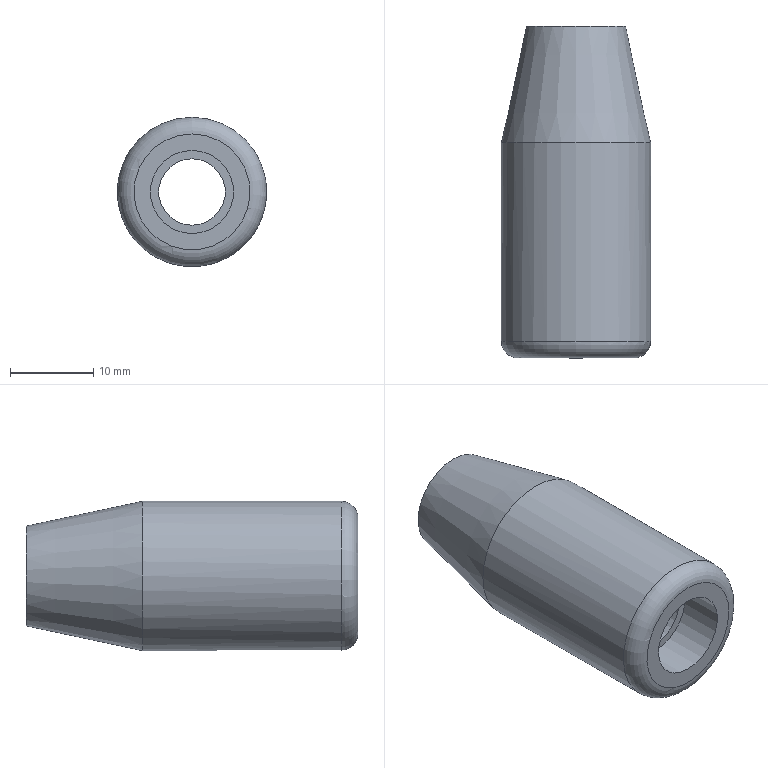Component | NX | HANDLE | 1 solid | 8 faces | box 17.95 x 39.9 x 17.95 mm | volume 6847 mm3 | plane 3 | cylinder 3 | cone 1 | torus 1 | commonest cylinder face diameters 17.952 x1 8 x1 10 x1
STEP:
#1=CARTESIAN_POINT('',(0.,0.,0.));
#2=DIRECTION('',(0.,0.,1.));
#3=DIRECTION('',(1.,0.,0.));
#4=AXIS2_PLACEMENT_3D('',#1,#2,#3);
#5=CARTESIAN_POINT('',(-0.,-194.8,71.));
#6=VERTEX_POINT('',#5);
#7=CARTESIAN_POINT('',(-0.,-194.8,67.));
#8=DIRECTION('',(0.,1.,0.));
#9=DIRECTION('',(0.,0.,1.));
#10=AXIS2_PLACEMENT_3D('',#7,#8,#9);
#11=CIRCLE('',#10,4.);
#12=CARTESIAN_POINT('',(-0.,-194.8,67.));
#13=DIRECTION('',(0.,1.,0.));
#14=DIRECTION('',(0.,0.,1.));
#15=AXIS2_PLACEMENT_3D('',#12,#13,#14);
#16=PLANE('',#15);
#17=CARTESIAN_POINT('',(0.,0.));
#18=DIRECTION('',(1.,0.));
#19=AXIS2_PLACEMENT_2D('',#17,#18);
#20=CIRCLE('',#19,4.);
#21=(GEOMETRIC_REPRESENTATION_CONTEXT(2)PARAMETRIC_REPRESENTATION_CONTEXT()REPRESENTATION_CONTEXT('',''));
#22=DEFINITIONAL_REPRESENTATION('',(#20),#21);
#23=PCURVE('',#16,#22);
#24=CARTESIAN_POINT('',(-0.,-188.739,67.));
#25=DIRECTION('',(0.,1.,0.));
#26=DIRECTION('',(0.,0.,1.));
#27=AXIS2_PLACEMENT_3D('',#24,#25,#26);
#28=CYLINDRICAL_SURFACE('',#27,4.);
#29=CARTESIAN_POINT('',(0.,-6.061));
#30=DIRECTION('',(1.,0.));
#31=VECTOR('',#30,1.);
#32=LINE('',#29,#31);
#33=(GEOMETRIC_REPRESENTATION_CONTEXT(2)PARAMETRIC_REPRESENTATION_CONTEXT()REPRESENTATION_CONTEXT('',''));
#34=DEFINITIONAL_REPRESENTATION('',(#32),#33);
#35=PCURVE('',#28,#34);
#36=SURFACE_CURVE('',#11,(#23,#35),.PCURVE_S1.);
#37=EDGE_CURVE('',#6,#6,#36,.T.);
#38=ORIENTED_EDGE('',*,*,#37,.F.);
#39=EDGE_LOOP('',(#38));
#40=FACE_BOUND('',#39,.T.);
#41=CARTESIAN_POINT('',(-0.,-194.8,61.));
#42=VERTEX_POINT('',#41);
#43=CARTESIAN_POINT('',(-0.,-194.8,67.));
#44=DIRECTION('',(0.,-1.,0.));
#45=DIRECTION('',(0.,0.,-1.));
#46=AXIS2_PLACEMENT_3D('',#43,#44,#45);
#47=CIRCLE('',#46,6.);
#48=CARTESIAN_POINT('',(-6.,0.));
#49=CARTESIAN_POINT('',(-6.,10.392));
#50=CARTESIAN_POINT('',(3.,5.196));
#51=CARTESIAN_POINT('',(12.,0.));
#52=CARTESIAN_POINT('',(3.,-5.196));
#53=CARTESIAN_POINT('',(-6.,-10.392));
#54=CARTESIAN_POINT('',(-6.,0.));
#55=(BOUNDED_CURVE()B_SPLINE_CURVE(2,(#48,#49,#50,#51,#52,#53,#54),.UNSPECIFIED.,.T.,.F.)B_SPLINE_CURVE_WITH_KNOTS((1,2,2,2,2,1),(-2.094,0.,2.094,4.189,6.283,8.378),.UNSPECIFIED.)CURVE()GEOMETRIC_REPRESENTATION_ITEM()RATIONAL_B_SPLINE_CURVE((1.,0.5,1.,0.5,1.,0.5,1.))REPRESENTATION_ITEM(''));
#56=(GEOMETRIC_REPRESENTATION_CONTEXT(2)PARAMETRIC_REPRESENTATION_CONTEXT()REPRESENTATION_CONTEXT('',''));
#57=DEFINITIONAL_REPRESENTATION('',(#55),#56);
#58=PCURVE('',#16,#57);
#59=CARTESIAN_POINT('',(-0.,-194.8,67.));
#60=DIRECTION('',(0.,-1.,0.));
#61=DIRECTION('',(0.,0.,-1.));
#62=AXIS2_PLACEMENT_3D('',#59,#60,#61);
#63=CONICAL_SURFACE('',#62,6.,0.2094);
#64=CARTESIAN_POINT('',(0.,0.));
#65=DIRECTION('',(1.,0.));
#66=VECTOR('',#65,1.);
#67=LINE('',#64,#66);
#68=(GEOMETRIC_REPRESENTATION_CONTEXT(2)PARAMETRIC_REPRESENTATION_CONTEXT()REPRESENTATION_CONTEXT('',''));
#69=DEFINITIONAL_REPRESENTATION('',(#67),#68);
#70=PCURVE('',#63,#69);
#71=SURFACE_CURVE('',#47,(#58,#70),.PCURVE_S1.);
#72=EDGE_CURVE('',#42,#42,#71,.T.);
#73=ORIENTED_EDGE('',*,*,#72,.F.);
#74=EDGE_LOOP('',(#73));
#75=FACE_BOUND('',#74,.T.);
#76=ADVANCED_FACE('',(#40,#75),#16,.T.);
#77=ORIENTED_EDGE('',*,*,#72,.T.);
#78=CARTESIAN_POINT('',(-0.,-208.8,58.024));
#79=VERTEX_POINT('',#78);
#80=CARTESIAN_POINT('',(-0.,-194.8,61.));
#81=CARTESIAN_POINT('',(-0.,-208.8,58.024));
#82=B_SPLINE_CURVE_WITH_KNOTS('',1,(#80,#81),.UNSPECIFIED.,.F.,.F.,(2,2),(0.,14.313),.PIECEWISE_BEZIER_KNOTS.);
#83=CARTESIAN_POINT('',(6.283,0.));
#84=DIRECTION('',(0.,1.));
#85=VECTOR('',#84,1.);
#86=LINE('',#83,#85);
#87=(GEOMETRIC_REPRESENTATION_CONTEXT(2)PARAMETRIC_REPRESENTATION_CONTEXT()REPRESENTATION_CONTEXT('',''));
#88=DEFINITIONAL_REPRESENTATION('',(#86),#87);
#89=PCURVE('',#63,#88);
#90=CARTESIAN_POINT('',(0.,0.));
#91=DIRECTION('',(0.,1.));
#92=VECTOR('',#91,1.);
#93=LINE('',#90,#92);
#94=(GEOMETRIC_REPRESENTATION_CONTEXT(2)PARAMETRIC_REPRESENTATION_CONTEXT()REPRESENTATION_CONTEXT('',''));
#95=DEFINITIONAL_REPRESENTATION('',(#93),#94);
#96=PCURVE('',#63,#95);
#97=SEAM_CURVE('',#82,(#89,#96),.PCURVE_S1.);
#98=EDGE_CURVE('',#42,#79,#97,.T.);
#99=ORIENTED_EDGE('',*,*,#98,.T.);
#100=CARTESIAN_POINT('',(-0.,-208.8,75.976));
#101=VERTEX_POINT('',#100);
#102=CARTESIAN_POINT('',(-0.,-208.8,67.));
#103=DIRECTION('',(0.,1.,0.));
#104=DIRECTION('',(0.,0.,-1.));
#105=AXIS2_PLACEMENT_3D('',#102,#103,#104);
#106=CIRCLE('',#105,8.976);
#107=CARTESIAN_POINT('',(6.283,14.));
#108=DIRECTION('',(-1.,0.));
#109=VECTOR('',#108,1.);
#110=LINE('',#107,#109);
#111=(GEOMETRIC_REPRESENTATION_CONTEXT(2)PARAMETRIC_REPRESENTATION_CONTEXT()REPRESENTATION_CONTEXT('',''));
#112=DEFINITIONAL_REPRESENTATION('',(#110),#111);
#113=PCURVE('',#63,#112);
#114=CARTESIAN_POINT('',(-0.,-234.7,67.));
#115=DIRECTION('',(0.,1.,0.));
#116=DIRECTION('',(0.,0.,1.));
#117=AXIS2_PLACEMENT_3D('',#114,#115,#116);
#118=CYLINDRICAL_SURFACE('',#117,8.976);
#119=CARTESIAN_POINT('',(3.142,25.9));
#120=DIRECTION('',(1.,0.));
#121=VECTOR('',#120,1.);
#122=LINE('',#119,#121);
#123=(GEOMETRIC_REPRESENTATION_CONTEXT(2)PARAMETRIC_REPRESENTATION_CONTEXT()REPRESENTATION_CONTEXT('',''));
#124=DEFINITIONAL_REPRESENTATION('',(#122),#123);
#125=PCURVE('',#118,#124);
#126=SURFACE_CURVE('',#106,(#113,#125),.PCURVE_S1.);
#127=EDGE_CURVE('',#79,#101,#126,.T.);
#128=ORIENTED_EDGE('',*,*,#127,.T.);
#129=CARTESIAN_POINT('',(-0.,-208.8,67.));
#130=DIRECTION('',(0.,1.,0.));
#131=DIRECTION('',(0.,0.,-1.));
#132=AXIS2_PLACEMENT_3D('',#129,#130,#131);
#133=CIRCLE('',#132,8.976);
#134=CARTESIAN_POINT('',(6.283,14.));
#135=DIRECTION('',(-1.,0.));
#136=VECTOR('',#135,1.);
#137=LINE('',#134,#136);
#138=(GEOMETRIC_REPRESENTATION_CONTEXT(2)PARAMETRIC_REPRESENTATION_CONTEXT()REPRESENTATION_CONTEXT('',''));
#139=DEFINITIONAL_REPRESENTATION('',(#137),#138);
#140=PCURVE('',#63,#139);
#141=CARTESIAN_POINT('',(-3.142,25.9));
#142=DIRECTION('',(1.,0.));
#143=VECTOR('',#142,1.);
#144=LINE('',#141,#143);
#145=(GEOMETRIC_REPRESENTATION_CONTEXT(2)PARAMETRIC_REPRESENTATION_CONTEXT()REPRESENTATION_CONTEXT('',''));
#146=DEFINITIONAL_REPRESENTATION('',(#144),#145);
#147=PCURVE('',#118,#146);
#148=SURFACE_CURVE('',#133,(#140,#147),.PCURVE_S1.);
#149=EDGE_CURVE('',#101,#79,#148,.T.);
#150=ORIENTED_EDGE('',*,*,#149,.T.);
#151=ORIENTED_EDGE('',*,*,#98,.F.);
#152=EDGE_LOOP('',(#77,#99,#128,#150,#151));
#153=FACE_BOUND('',#152,.T.);
#154=ADVANCED_FACE('',(#153),#63,.T.);
#155=CARTESIAN_POINT('',(-0.,-232.7,75.976));
#156=VERTEX_POINT('',#155);
#157=CARTESIAN_POINT('',(-0.,-232.7,67.));
#158=DIRECTION('',(0.,1.,0.));
#159=DIRECTION('',(0.,0.,1.));
#160=AXIS2_PLACEMENT_3D('',#157,#158,#159);
#161=CIRCLE('',#160,8.976);
#162=CARTESIAN_POINT('',(0.,2.));
#163=DIRECTION('',(1.,0.));
#164=VECTOR('',#163,1.);
#165=LINE('',#162,#164);
#166=(GEOMETRIC_REPRESENTATION_CONTEXT(2)PARAMETRIC_REPRESENTATION_CONTEXT()REPRESENTATION_CONTEXT('',''));
#167=DEFINITIONAL_REPRESENTATION('',(#165),#166);
#168=PCURVE('',#118,#167);
#169=CARTESIAN_POINT('',(-0.,-232.7,67.));
#170=DIRECTION('',(0.,1.,0.));
#171=DIRECTION('',(0.,0.,1.));
#172=AXIS2_PLACEMENT_3D('',#169,#170,#171);
#173=TOROIDAL_SURFACE('',#172,6.976,2.);
#174=CARTESIAN_POINT('',(0.,6.283));
#175=DIRECTION('',(1.,0.));
#176=VECTOR('',#175,1.);
#177=LINE('',#174,#176);
#178=(GEOMETRIC_REPRESENTATION_CONTEXT(2)PARAMETRIC_REPRESENTATION_CONTEXT()REPRESENTATION_CONTEXT('',''));
#179=DEFINITIONAL_REPRESENTATION('',(#177),#178);
#180=PCURVE('',#173,#179);
#181=SURFACE_CURVE('',#161,(#168,#180),.PCURVE_S1.);
#182=EDGE_CURVE('',#156,#156,#181,.T.);
#183=ORIENTED_EDGE('',*,*,#182,.T.);
#184=CARTESIAN_POINT('',(-0.,-232.7,75.976));
#185=CARTESIAN_POINT('',(-0.,-208.8,75.976));
#186=B_SPLINE_CURVE_WITH_KNOTS('',1,(#184,#185),.UNSPECIFIED.,.F.,.F.,(2,2),(2.,25.9),.PIECEWISE_BEZIER_KNOTS.);
#187=CARTESIAN_POINT('',(6.283,0.));
#188=DIRECTION('',(0.,1.));
#189=VECTOR('',#188,1.);
#190=LINE('',#187,#189);
#191=(GEOMETRIC_REPRESENTATION_CONTEXT(2)PARAMETRIC_REPRESENTATION_CONTEXT()REPRESENTATION_CONTEXT('',''));
#192=DEFINITIONAL_REPRESENTATION('',(#190),#191);
#193=PCURVE('',#118,#192);
#194=CARTESIAN_POINT('',(0.,0.));
#195=DIRECTION('',(0.,1.));
#196=VECTOR('',#195,1.);
#197=LINE('',#194,#196);
#198=(GEOMETRIC_REPRESENTATION_CONTEXT(2)PARAMETRIC_REPRESENTATION_CONTEXT()REPRESENTATION_CONTEXT('',''));
#199=DEFINITIONAL_REPRESENTATION('',(#197),#198);
#200=PCURVE('',#118,#199);
#201=SEAM_CURVE('',#186,(#193,#200),.PCURVE_S1.);
#202=EDGE_CURVE('',#156,#101,#201,.T.);
#203=ORIENTED_EDGE('',*,*,#202,.T.);
#204=ORIENTED_EDGE('',*,*,#127,.F.);
#205=ORIENTED_EDGE('',*,*,#149,.F.);
#206=ORIENTED_EDGE('',*,*,#202,.F.);
#207=EDGE_LOOP('',(#183,#203,#204,#205,#206));
#208=FACE_BOUND('',#207,.T.);
#209=ADVANCED_FACE('',(#208),#118,.T.);
#210=CARTESIAN_POINT('',(-0.,-234.7,73.976));
#211=VERTEX_POINT('',#210);
#212=CARTESIAN_POINT('',(-0.,-234.7,67.));
#213=DIRECTION('',(0.,-1.,0.));
#214=DIRECTION('',(0.,0.,1.));
#215=AXIS2_PLACEMENT_3D('',#212,#213,#214);
#216=CIRCLE('',#215,6.976);
#217=CARTESIAN_POINT('',(-0.,-234.7,67.));
#218=DIRECTION('',(0.,1.,0.));
#219=DIRECTION('',(0.,0.,1.));
#220=AXIS2_PLACEMENT_3D('',#217,#218,#219);
#221=PLANE('',#220);
#222=CARTESIAN_POINT('',(6.976,0.));
#223=CARTESIAN_POINT('',(6.976,-12.082));
#224=CARTESIAN_POINT('',(-3.488,-6.041));
#225=CARTESIAN_POINT('',(-13.952,-0.));
#226=CARTESIAN_POINT('',(-3.488,6.041));
#227=CARTESIAN_POINT('',(6.976,12.082));
#228=CARTESIAN_POINT('',(6.976,0.));
#229=(BOUNDED_CURVE()B_SPLINE_CURVE(2,(#222,#223,#224,#225,#226,#227,#228),.UNSPECIFIED.,.T.,.F.)B_SPLINE_CURVE_WITH_KNOTS((1,2,2,2,2,1),(-2.094,0.,2.094,4.189,6.283,8.378),.UNSPECIFIED.)CURVE()GEOMETRIC_REPRESENTATION_ITEM()RATIONAL_B_SPLINE_CURVE((1.,0.5,1.,0.5,1.,0.5,1.))REPRESENTATION_ITEM(''));
#230=(GEOMETRIC_REPRESENTATION_CONTEXT(2)PARAMETRIC_REPRESENTATION_CONTEXT()REPRESENTATION_CONTEXT('',''));
#231=DEFINITIONAL_REPRESENTATION('',(#229),#230);
#232=PCURVE('',#221,#231);
#233=CARTESIAN_POINT('',(6.283,4.712));
#234=DIRECTION('',(-1.,0.));
#235=VECTOR('',#234,1.);
#236=LINE('',#233,#235);
#237=(GEOMETRIC_REPRESENTATION_CONTEXT(2)PARAMETRIC_REPRESENTATION_CONTEXT()REPRESENTATION_CONTEXT('',''));
#238=DEFINITIONAL_REPRESENTATION('',(#236),#237);
#239=PCURVE('',#173,#238);
#240=SURFACE_CURVE('',#216,(#232,#239),.PCURVE_S1.);
#241=EDGE_CURVE('',#211,#211,#240,.T.);
#242=ORIENTED_EDGE('',*,*,#241,.T.);
#243=EDGE_LOOP('',(#242));
#244=FACE_BOUND('',#243,.T.);
#245=CARTESIAN_POINT('',(-0.,-234.7,72.));
#246=VERTEX_POINT('',#245);
#247=CARTESIAN_POINT('',(-0.,-234.7,67.));
#248=DIRECTION('',(0.,1.,0.));
#249=DIRECTION('',(0.,0.,1.));
#250=AXIS2_PLACEMENT_3D('',#247,#248,#249);
#251=CIRCLE('',#250,5.);
#252=CARTESIAN_POINT('',(0.,0.));
#253=DIRECTION('',(1.,0.));
#254=AXIS2_PLACEMENT_2D('',#252,#253);
#255=CIRCLE('',#254,5.);
#256=(GEOMETRIC_REPRESENTATION_CONTEXT(2)PARAMETRIC_REPRESENTATION_CONTEXT()REPRESENTATION_CONTEXT('',''));
#257=DEFINITIONAL_REPRESENTATION('',(#255),#256);
#258=PCURVE('',#221,#257);
#259=CARTESIAN_POINT('',(-0.,-234.7,67.));
#260=DIRECTION('',(0.,1.,0.));
#261=DIRECTION('',(0.,0.,1.));
#262=AXIS2_PLACEMENT_3D('',#259,#260,#261);
#263=CYLINDRICAL_SURFACE('',#262,5.);
#264=CARTESIAN_POINT('',(0.,0.));
#265=DIRECTION('',(1.,0.));
#266=VECTOR('',#265,1.);
#267=LINE('',#264,#266);
#268=(GEOMETRIC_REPRESENTATION_CONTEXT(2)PARAMETRIC_REPRESENTATION_CONTEXT()REPRESENTATION_CONTEXT('',''));
#269=DEFINITIONAL_REPRESENTATION('',(#267),#268);
#270=PCURVE('',#263,#269);
#271=SURFACE_CURVE('',#251,(#258,#270),.PCURVE_S1.);
#272=EDGE_CURVE('',#246,#246,#271,.T.);
#273=ORIENTED_EDGE('',*,*,#272,.T.);
#274=EDGE_LOOP('',(#273));
#275=FACE_BOUND('',#274,.T.);
#276=ADVANCED_FACE('',(#244,#275),#221,.F.);
#277=ORIENTED_EDGE('',*,*,#37,.F.);
#278=CARTESIAN_POINT('',(-0.,-229.2,71.));
#279=VERTEX_POINT('',#278);
#280=CARTESIAN_POINT('',(-0.,-229.2,71.));
#281=CARTESIAN_POINT('',(-0.,-194.8,71.));
#282=B_SPLINE_CURVE_WITH_KNOTS('',1,(#280,#281),.UNSPECIFIED.,.F.,.F.,(2,2),(-40.461,-6.061),.PIECEWISE_BEZIER_KNOTS.);
#283=CARTESIAN_POINT('',(0.,0.));
#284=DIRECTION('',(0.,1.));
#285=VECTOR('',#284,1.);
#286=LINE('',#283,#285);
#287=(GEOMETRIC_REPRESENTATION_CONTEXT(2)PARAMETRIC_REPRESENTATION_CONTEXT()REPRESENTATION_CONTEXT('',''));
#288=DEFINITIONAL_REPRESENTATION('',(#286),#287);
#289=PCURVE('',#28,#288);
#290=CARTESIAN_POINT('',(6.283,0.));
#291=DIRECTION('',(0.,1.));
#292=VECTOR('',#291,1.);
#293=LINE('',#290,#292);
#294=(GEOMETRIC_REPRESENTATION_CONTEXT(2)PARAMETRIC_REPRESENTATION_CONTEXT()REPRESENTATION_CONTEXT('',''));
#295=DEFINITIONAL_REPRESENTATION('',(#293),#294);
#296=PCURVE('',#28,#295);
#297=SEAM_CURVE('',#282,(#289,#296),.PCURVE_S1.);
#298=EDGE_CURVE('',#279,#6,#297,.T.);
#299=ORIENTED_EDGE('',*,*,#298,.F.);
#300=CARTESIAN_POINT('',(-0.,-229.2,67.));
#301=DIRECTION('',(0.,-1.,0.));
#302=DIRECTION('',(0.,0.,1.));
#303=AXIS2_PLACEMENT_3D('',#300,#301,#302);
#304=CIRCLE('',#303,4.);
#305=CARTESIAN_POINT('',(6.283,-40.461));
#306=DIRECTION('',(-1.,0.));
#307=VECTOR('',#306,1.);
#308=LINE('',#305,#307);
#309=(GEOMETRIC_REPRESENTATION_CONTEXT(2)PARAMETRIC_REPRESENTATION_CONTEXT()REPRESENTATION_CONTEXT('',''));
#310=DEFINITIONAL_REPRESENTATION('',(#308),#309);
#311=PCURVE('',#28,#310);
#312=CARTESIAN_POINT('',(-0.,-229.2,67.));
#313=DIRECTION('',(0.,1.,0.));
#314=DIRECTION('',(0.,0.,1.));
#315=AXIS2_PLACEMENT_3D('',#312,#313,#314);
#316=PLANE('',#315);
#317=CARTESIAN_POINT('',(4.,0.));
#318=CARTESIAN_POINT('',(4.,-6.928));
#319=CARTESIAN_POINT('',(-2.,-3.464));
#320=CARTESIAN_POINT('',(-8.,-0.));
#321=CARTESIAN_POINT('',(-2.,3.464));
#322=CARTESIAN_POINT('',(4.,6.928));
#323=CARTESIAN_POINT('',(4.,0.));
#324=(BOUNDED_CURVE()B_SPLINE_CURVE(2,(#317,#318,#319,#320,#321,#322,#323),.UNSPECIFIED.,.T.,.F.)B_SPLINE_CURVE_WITH_KNOTS((1,2,2,2,2,1),(-2.094,0.,2.094,4.189,6.283,8.378),.UNSPECIFIED.)CURVE()GEOMETRIC_REPRESENTATION_ITEM()RATIONAL_B_SPLINE_CURVE((1.,0.5,1.,0.5,1.,0.5,1.))REPRESENTATION_ITEM(''));
#325=(GEOMETRIC_REPRESENTATION_CONTEXT(2)PARAMETRIC_REPRESENTATION_CONTEXT()REPRESENTATION_CONTEXT('',''));
#326=DEFINITIONAL_REPRESENTATION('',(#324),#325);
#327=PCURVE('',#316,#326);
#328=SURFACE_CURVE('',#304,(#311,#327),.PCURVE_S1.);
#329=EDGE_CURVE('',#279,#279,#328,.T.);
#330=ORIENTED_EDGE('',*,*,#329,.F.);
#331=ORIENTED_EDGE('',*,*,#298,.T.);
#332=EDGE_LOOP('',(#277,#299,#330,#331));
#333=FACE_BOUND('',#332,.F.);
#334=ADVANCED_FACE('',(#333),#28,.F.);
#335=ORIENTED_EDGE('',*,*,#329,.F.);
#336=EDGE_LOOP('',(#335));
#337=FACE_BOUND('',#336,.T.);
#338=CARTESIAN_POINT('',(-0.,-229.2,72.));
#339=VERTEX_POINT('',#338);
#340=CARTESIAN_POINT('',(-0.,-229.2,67.));
#341=DIRECTION('',(0.,-1.,0.));
#342=DIRECTION('',(0.,0.,1.));
#343=AXIS2_PLACEMENT_3D('',#340,#341,#342);
#344=CIRCLE('',#343,5.);
#345=CARTESIAN_POINT('',(5.,0.));
#346=CARTESIAN_POINT('',(5.,-8.66));
#347=CARTESIAN_POINT('',(-2.5,-4.33));
#348=CARTESIAN_POINT('',(-10.,-0.));
#349=CARTESIAN_POINT('',(-2.5,4.33));
#350=CARTESIAN_POINT('',(5.,8.66));
#351=CARTESIAN_POINT('',(5.,0.));
#352=(BOUNDED_CURVE()B_SPLINE_CURVE(2,(#345,#346,#347,#348,#349,#350,#351),.UNSPECIFIED.,.T.,.F.)B_SPLINE_CURVE_WITH_KNOTS((1,2,2,2,2,1),(-2.094,0.,2.094,4.189,6.283,8.378),.UNSPECIFIED.)CURVE()GEOMETRIC_REPRESENTATION_ITEM()RATIONAL_B_SPLINE_CURVE((1.,0.5,1.,0.5,1.,0.5,1.))REPRESENTATION_ITEM(''));
#353=(GEOMETRIC_REPRESENTATION_CONTEXT(2)PARAMETRIC_REPRESENTATION_CONTEXT()REPRESENTATION_CONTEXT('',''));
#354=DEFINITIONAL_REPRESENTATION('',(#352),#353);
#355=PCURVE('',#316,#354);
#356=CARTESIAN_POINT('',(6.283,5.5));
#357=DIRECTION('',(-1.,0.));
#358=VECTOR('',#357,1.);
#359=LINE('',#356,#358);
#360=(GEOMETRIC_REPRESENTATION_CONTEXT(2)PARAMETRIC_REPRESENTATION_CONTEXT()REPRESENTATION_CONTEXT('',''));
#361=DEFINITIONAL_REPRESENTATION('',(#359),#360);
#362=PCURVE('',#263,#361);
#363=SURFACE_CURVE('',#344,(#355,#362),.PCURVE_S1.);
#364=EDGE_CURVE('',#339,#339,#363,.T.);
#365=ORIENTED_EDGE('',*,*,#364,.T.);
#366=EDGE_LOOP('',(#365));
#367=FACE_BOUND('',#366,.T.);
#368=ADVANCED_FACE('',(#337,#367),#316,.F.);
#369=ORIENTED_EDGE('',*,*,#364,.T.);
#370=CARTESIAN_POINT('',(-0.,-234.7,72.));
#371=CARTESIAN_POINT('',(-0.,-229.2,72.));
#372=B_SPLINE_CURVE_WITH_KNOTS('',1,(#370,#371),.UNSPECIFIED.,.F.,.F.,(2,2),(0.,5.5),.PIECEWISE_BEZIER_KNOTS.);
#373=CARTESIAN_POINT('',(0.,0.));
#374=DIRECTION('',(0.,1.));
#375=VECTOR('',#374,1.);
#376=LINE('',#373,#375);
#377=(GEOMETRIC_REPRESENTATION_CONTEXT(2)PARAMETRIC_REPRESENTATION_CONTEXT()REPRESENTATION_CONTEXT('',''));
#378=DEFINITIONAL_REPRESENTATION('',(#376),#377);
#379=PCURVE('',#263,#378);
#380=CARTESIAN_POINT('',(6.283,0.));
#381=DIRECTION('',(0.,1.));
#382=VECTOR('',#381,1.);
#383=LINE('',#380,#382);
#384=(GEOMETRIC_REPRESENTATION_CONTEXT(2)PARAMETRIC_REPRESENTATION_CONTEXT()REPRESENTATION_CONTEXT('',''));
#385=DEFINITIONAL_REPRESENTATION('',(#383),#384);
#386=PCURVE('',#263,#385);
#387=SEAM_CURVE('',#372,(#379,#386),.PCURVE_S1.);
#388=EDGE_CURVE('',#246,#339,#387,.T.);
#389=ORIENTED_EDGE('',*,*,#388,.F.);
#390=ORIENTED_EDGE('',*,*,#272,.T.);
#391=ORIENTED_EDGE('',*,*,#388,.T.);
#392=EDGE_LOOP('',(#369,#389,#390,#391));
#393=FACE_BOUND('',#392,.F.);
#394=ADVANCED_FACE('',(#393),#263,.F.);
#395=ORIENTED_EDGE('',*,*,#241,.F.);
#396=CARTESIAN_POINT('',(-0.,-234.7,73.976));
#397=CARTESIAN_POINT('',(-0.,-234.7,74.51));
#398=CARTESIAN_POINT('',(-0.,-234.53,75.031));
#399=CARTESIAN_POINT('',(-0.,-234.204,75.48));
#400=CARTESIAN_POINT('',(-0.,-233.755,75.806));
#401=CARTESIAN_POINT('',(-0.,-233.235,75.976));
#402=CARTESIAN_POINT('',(-0.,-232.7,75.976));
#403=(BOUNDED_CURVE()B_SPLINE_CURVE(6,(#396,#397,#398,#399,#400,#401,#402),.UNSPECIFIED.,.F.,.F.)B_SPLINE_CURVE_WITH_KNOTS((7,7),(4.712,6.283),.PIECEWISE_BEZIER_KNOTS.)CURVE()GEOMETRIC_REPRESENTATION_ITEM()RATIONAL_B_SPLINE_CURVE((1.031,1.01,0.9979,0.994,0.9979,1.01,1.031))REPRESENTATION_ITEM(''));
#404=CARTESIAN_POINT('',(6.283,0.));
#405=DIRECTION('',(0.,1.));
#406=VECTOR('',#405,1.);
#407=LINE('',#404,#406);
#408=(GEOMETRIC_REPRESENTATION_CONTEXT(2)PARAMETRIC_REPRESENTATION_CONTEXT()REPRESENTATION_CONTEXT('',''));
#409=DEFINITIONAL_REPRESENTATION('',(#407),#408);
#410=PCURVE('',#173,#409);
#411=CARTESIAN_POINT('',(0.,0.));
#412=DIRECTION('',(0.,1.));
#413=VECTOR('',#412,1.);
#414=LINE('',#411,#413);
#415=(GEOMETRIC_REPRESENTATION_CONTEXT(2)PARAMETRIC_REPRESENTATION_CONTEXT()REPRESENTATION_CONTEXT('',''));
#416=DEFINITIONAL_REPRESENTATION('',(#414),#415);
#417=PCURVE('',#173,#416);
#418=SEAM_CURVE('',#403,(#410,#417),.PCURVE_S1.);
#419=EDGE_CURVE('',#211,#156,#418,.T.);
#420=ORIENTED_EDGE('',*,*,#419,.T.);
#421=ORIENTED_EDGE('',*,*,#182,.F.);
#422=ORIENTED_EDGE('',*,*,#419,.F.);
#423=EDGE_LOOP('',(#395,#420,#421,#422));
#424=FACE_BOUND('',#423,.T.);
#425=ADVANCED_FACE('',(#424),#173,.T.);
#426=CLOSED_SHELL('',(#76,#154,#209,#276,#334,#368,#394,#425));
#427=MANIFOLD_SOLID_BREP('',#426);
#428=(LENGTH_UNIT()NAMED_UNIT(*)SI_UNIT(.MILLI.,.METRE.));
#429=UNCERTAINTY_MEASURE_WITH_UNIT(LENGTH_MEASURE(0.00001),#428,'','');
#430=(NAMED_UNIT(*)PLANE_ANGLE_UNIT()SI_UNIT($,.RADIAN.));
#431=(NAMED_UNIT(*)SI_UNIT($,.STERADIAN.)SOLID_ANGLE_UNIT());
#432=(GEOMETRIC_REPRESENTATION_CONTEXT(3)GLOBAL_UNCERTAINTY_ASSIGNED_CONTEXT((#429))GLOBAL_UNIT_ASSIGNED_CONTEXT((#428,#430,#431))REPRESENTATION_CONTEXT('',''));
#433=ADVANCED_BREP_SHAPE_REPRESENTATION('',(#4,#427),#432);